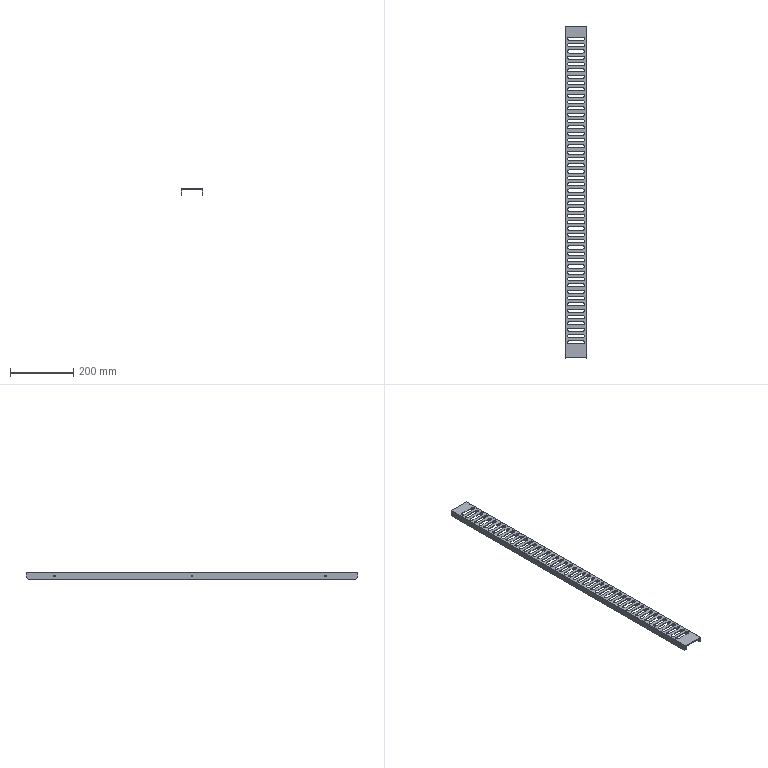Component | SolidWorks | WireDuct2-1 | 1 solid | 271 faces | box 68 x 1050 x 20 mm | volume 168161 mm3 | cylinder 163 | plane 108 | commonest cylinder face diameters 9.991 x147 6 x12 20 x4
build123d program:
from build123d import *

# Parameters (mm, degrees)
BOSS_EXTRUDE1_DEPTH       = 525
BOSS_EXTRUDE1_DEPTH_BACK  = 525
SIZE_MM_DOWEL_PIN_HOLE1_D = 6
FILLET1_R                 = 10
CUT_EXTRUDE1_DEPTH        = 10


with BuildPart() as part:
    # Sketch1 → Boss-Extrude1 (new, two sides: drawn at the far end of the back side and taken through both)
    with BuildSketch(Plane(origin=(0, 0, 0), x_dir=(1, 0, 0), z_dir=(0, 1, 0)).offset(-BOSS_EXTRUDE1_DEPTH_BACK)):
        Polygon((32, 10), (32, -8), (-32, -8), (-32, 10), (-34, 10), (-34, -10), (34, -10), (34, 10), align=None)
    extrude(amount=BOSS_EXTRUDE1_DEPTH + BOSS_EXTRUDE1_DEPTH_BACK)

    # Size mm Dowel Pin Hole1 (through all)
    with Locations(Plane(origin=(34, 0, 0), x_dir=(0, 0, -1), z_dir=(1, 0, 0))):
        with Locations((0, 435.363), (0, 0), (0, -423.324)):
            Hole(SIZE_MM_DOWEL_PIN_HOLE1_D / 2)

    # Fillet1
    fillet1_edges = [part.edges().sort_by_distance(p)[0] for p in [
        (-33, -525, -10),
        (33, 525, -10),
        (-33, 525, -10),
        (33, -525, -10),
    ]]
    fillet(fillet1_edges, radius=FILLET1_R)

    # Sketch5 → Cut-Extrude1 (cut)
    with BuildSketch(Plane.XY.offset(10)):
        with BuildLine():
            Line((-21.471, 489.584), (21.471, 489.584))
            ThreePointArc((21.471, 489.584), (26.467, 484.588), (21.471, 479.593))
            Line((21.471, 479.593), (-21.471, 479.593))
            ThreePointArc((-21.471, 479.593), (-26.467, 484.588), (-21.471, 489.584))
        make_face()
        with BuildLine():
            Line((-21.471, 469.584), (21.471, 469.584))
            ThreePointArc((21.471, 469.584), (26.467, 464.588), (21.471, 459.593))
            Line((21.471, 459.593), (-21.471, 459.593))
            ThreePointArc((-21.471, 459.593), (-26.467, 464.588), (-21.471, 469.584))
        make_face()
        with BuildLine():
            Line((-21.471, 449.584), (21.471, 449.584))
            ThreePointArc((21.471, 449.584), (26.467, 444.588), (21.471, 439.593))
            Line((21.471, 439.593), (-21.471, 439.593))
            ThreePointArc((-21.471, 439.593), (-26.467, 444.588), (-21.471, 449.584))
        make_face()
        with BuildLine():
            Line((-21.471, 429.584), (21.471, 429.584))
            ThreePointArc((21.471, 429.584), (26.467, 424.588), (21.471, 419.593))
            Line((21.471, 419.593), (-21.471, 419.593))
            ThreePointArc((-21.471, 419.593), (-26.467, 424.588), (-21.471, 429.584))
        make_face()
        with BuildLine():
            Line((-21.471, 409.584), (21.471, 409.584))
            ThreePointArc((21.471, 409.584), (26.467, 404.588), (21.471, 399.593))
            Line((21.471, 399.593), (-21.471, 399.593))
            ThreePointArc((-21.471, 399.593), (-26.467, 404.588), (-21.471, 409.584))
        make_face()
        with BuildLine():
            Line((-21.471, 389.584), (21.471, 389.584))
            ThreePointArc((21.471, 389.584), (26.467, 384.588), (21.471, 379.593))
            Line((21.471, 379.593), (-21.471, 379.593))
            ThreePointArc((-21.471, 379.593), (-26.467, 384.588), (-21.471, 389.584))
        make_face()
        with BuildLine():
            Line((-21.471, 369.584), (21.471, 369.584))
            ThreePointArc((21.471, 369.584), (26.467, 364.588), (21.471, 359.593))
            Line((21.471, 359.593), (-21.471, 359.593))
            ThreePointArc((-21.471, 359.593), (-26.467, 364.588), (-21.471, 369.584))
        make_face()
        with BuildLine():
            Line((-21.471, 349.584), (21.471, 349.584))
            ThreePointArc((21.471, 349.584), (26.467, 344.588), (21.471, 339.593))
            Line((21.471, 339.593), (-21.471, 339.593))
            ThreePointArc((-21.471, 339.593), (-26.467, 344.588), (-21.471, 349.584))
        make_face()
        with BuildLine():
            Line((-21.471, 329.584), (21.471, 329.584))
            ThreePointArc((21.471, 329.584), (26.467, 324.588), (21.471, 319.593))
            Line((21.471, 319.593), (-21.471, 319.593))
            ThreePointArc((-21.471, 319.593), (-26.467, 324.588), (-21.471, 329.584))
        make_face()
        with BuildLine():
            Line((-21.471, 309.584), (21.471, 309.584))
            ThreePointArc((21.471, 309.584), (26.467, 304.588), (21.471, 299.593))
            Line((21.471, 299.593), (-21.471, 299.593))
            ThreePointArc((-21.471, 299.593), (-26.467, 304.588), (-21.471, 309.584))
        make_face()
        with BuildLine():
            Line((-21.471, 289.584), (21.471, 289.584))
            ThreePointArc((21.471, 289.584), (26.467, 284.588), (21.471, 279.593))
            Line((21.471, 279.593), (-21.471, 279.593))
            ThreePointArc((-21.471, 279.593), (-26.467, 284.588), (-21.471, 289.584))
        make_face()
        with BuildLine():
            Line((-21.471, 269.584), (21.471, 269.584))
            ThreePointArc((21.471, 269.584), (26.467, 264.588), (21.471, 259.593))
            Line((21.471, 259.593), (-21.471, 259.593))
            ThreePointArc((-21.471, 259.593), (-26.467, 264.588), (-21.471, 269.584))
        make_face()
        with BuildLine():
            Line((-21.471, 249.584), (21.471, 249.584))
            ThreePointArc((21.471, 249.584), (26.467, 244.588), (21.471, 239.593))
            Line((21.471, 239.593), (-21.471, 239.593))
            ThreePointArc((-21.471, 239.593), (-26.467, 244.588), (-21.471, 249.584))
        make_face()
        with BuildLine():
            Line((-21.471, 229.584), (21.471, 229.584))
            ThreePointArc((21.471, 229.584), (26.467, 224.588), (21.471, 219.593))
            Line((21.471, 219.593), (-21.471, 219.593))
            ThreePointArc((-21.471, 219.593), (-26.467, 224.588), (-21.471, 229.584))
        make_face()
        with BuildLine():
            Line((-21.471, 209.584), (21.471, 209.584))
            ThreePointArc((21.471, 209.584), (26.467, 204.588), (21.471, 199.593))
            Line((21.471, 199.593), (-21.471, 199.593))
            ThreePointArc((-21.471, 199.593), (-26.467, 204.588), (-21.471, 209.584))
        make_face()
        with BuildLine():
            Line((-21.471, 189.584), (21.471, 189.584))
            ThreePointArc((21.471, 189.584), (26.467, 184.588), (21.471, 179.593))
            Line((21.471, 179.593), (-21.471, 179.593))
            ThreePointArc((-21.471, 179.593), (-26.467, 184.588), (-21.471, 189.584))
        make_face()
        with BuildLine():
            Line((-21.471, 169.584), (21.471, 169.584))
            ThreePointArc((21.471, 169.584), (26.467, 164.588), (21.471, 159.593))
            Line((21.471, 159.593), (-21.471, 159.593))
            ThreePointArc((-21.471, 159.593), (-26.467, 164.588), (-21.471, 169.584))
        make_face()
        with BuildLine():
            Line((-21.471, 149.584), (21.471, 149.584))
            ThreePointArc((21.471, 149.584), (26.467, 144.588), (21.471, 139.593))
            Line((21.471, 139.593), (-21.471, 139.593))
            ThreePointArc((-21.471, 139.593), (-26.467, 144.588), (-21.471, 149.584))
        make_face()
        with BuildLine():
            Line((-21.471, 129.584), (21.471, 129.584))
            ThreePointArc((21.471, 129.584), (26.467, 124.588), (21.471, 119.593))
            Line((21.471, 119.593), (-21.471, 119.593))
            ThreePointArc((-21.471, 119.593), (-26.467, 124.588), (-21.471, 129.584))
        make_face()
        with BuildLine():
            Line((-21.471, 109.584), (21.471, 109.584))
            ThreePointArc((21.471, 109.584), (26.467, 104.588), (21.471, 99.593))
            Line((21.471, 99.593), (-21.471, 99.593))
            ThreePointArc((-21.471, 99.593), (-26.467, 104.588), (-21.471, 109.584))
        make_face()
        with BuildLine():
            Line((-21.471, 89.584), (21.471, 89.584))
            ThreePointArc((21.471, 89.584), (26.467, 84.588), (21.471, 79.593))
            Line((21.471, 79.593), (-21.471, 79.593))
            ThreePointArc((-21.471, 79.593), (-26.467, 84.588), (-21.471, 89.584))
        make_face()
        with BuildLine():
            Line((-21.471, 69.584), (21.471, 69.584))
            ThreePointArc((21.471, 69.584), (26.467, 64.588), (21.471, 59.593))
            Line((21.471, 59.593), (-21.471, 59.593))
            ThreePointArc((-21.471, 59.593), (-26.467, 64.588), (-21.471, 69.584))
        make_face()
        with BuildLine():
            Line((-21.471, 49.584), (21.471, 49.584))
            ThreePointArc((21.471, 49.584), (26.467, 44.588), (21.471, 39.593))
            Line((21.471, 39.593), (-21.471, 39.593))
            ThreePointArc((-21.471, 39.593), (-26.467, 44.588), (-21.471, 49.584))
        make_face()
        with BuildLine():
            Line((-21.471, 29.584), (21.471, 29.584))
            ThreePointArc((21.471, 29.584), (26.467, 24.588), (21.471, 19.593))
            Line((21.471, 19.593), (-21.471, 19.593))
            ThreePointArc((-21.471, 19.593), (-26.467, 24.588), (-21.471, 29.584))
        make_face()
        with BuildLine():
            Line((-21.471, 9.584), (21.471, 9.584))
            ThreePointArc((21.471, 9.584), (26.467, 4.588), (21.471, -0.4072))
            Line((21.471, -0.4072), (-21.471, -0.4072))
            ThreePointArc((-21.471, -0.4072), (-26.467, 4.588), (-21.471, 9.584))
        make_face()
        with BuildLine():
            Line((-21.471, -10.416), (21.471, -10.416))
            ThreePointArc((21.471, -10.416), (26.467, -15.412), (21.471, -20.407))
            Line((21.471, -20.407), (-21.471, -20.407))
            ThreePointArc((-21.471, -20.407), (-26.467, -15.412), (-21.471, -10.416))
        make_face()
        with BuildLine():
            Line((-21.471, -30.416), (21.471, -30.416))
            ThreePointArc((21.471, -30.416), (26.467, -35.412), (21.471, -40.407))
            Line((21.471, -40.407), (-21.471, -40.407))
            ThreePointArc((-21.471, -40.407), (-26.467, -35.412), (-21.471, -30.416))
        make_face()
        with BuildLine():
            Line((-21.471, -50.416), (21.471, -50.416))
            ThreePointArc((21.471, -50.416), (26.467, -55.412), (21.471, -60.407))
            Line((21.471, -60.407), (-21.471, -60.407))
            ThreePointArc((-21.471, -60.407), (-26.467, -55.412), (-21.471, -50.416))
        make_face()
        with BuildLine():
            Line((-21.471, -70.416), (21.471, -70.416))
            ThreePointArc((21.471, -70.416), (26.467, -75.412), (21.471, -80.407))
            Line((21.471, -80.407), (-21.471, -80.407))
            ThreePointArc((-21.471, -80.407), (-26.467, -75.412), (-21.471, -70.416))
        make_face()
        with BuildLine():
            Line((-21.471, -90.416), (21.471, -90.416))
            ThreePointArc((21.471, -90.416), (26.467, -95.412), (21.471, -100.407))
            Line((21.471, -100.407), (-21.471, -100.407))
            ThreePointArc((-21.471, -100.407), (-26.467, -95.412), (-21.471, -90.416))
        make_face()
        with BuildLine():
            Line((-21.471, -110.416), (21.471, -110.416))
            ThreePointArc((21.471, -110.416), (26.467, -115.412), (21.471, -120.407))
            Line((21.471, -120.407), (-21.471, -120.407))
            ThreePointArc((-21.471, -120.407), (-26.467, -115.412), (-21.471, -110.416))
        make_face()
        with BuildLine():
            Line((-21.471, -130.416), (21.471, -130.416))
            ThreePointArc((21.471, -130.416), (26.467, -135.412), (21.471, -140.407))
            Line((21.471, -140.407), (-21.471, -140.407))
            ThreePointArc((-21.471, -140.407), (-26.467, -135.412), (-21.471, -130.416))
        make_face()
        with BuildLine():
            Line((-21.471, -150.416), (21.471, -150.416))
            ThreePointArc((21.471, -150.416), (26.467, -155.412), (21.471, -160.407))
            Line((21.471, -160.407), (-21.471, -160.407))
            ThreePointArc((-21.471, -160.407), (-26.467, -155.412), (-21.471, -150.416))
        make_face()
        with BuildLine():
            Line((-21.471, -170.416), (21.471, -170.416))
            ThreePointArc((21.471, -170.416), (26.467, -175.412), (21.471, -180.407))
            Line((21.471, -180.407), (-21.471, -180.407))
            ThreePointArc((-21.471, -180.407), (-26.467, -175.412), (-21.471, -170.416))
        make_face()
        with BuildLine():
            Line((-21.471, -190.416), (21.471, -190.416))
            ThreePointArc((21.471, -190.416), (26.467, -195.412), (21.471, -200.407))
            Line((21.471, -200.407), (-21.471, -200.407))
            ThreePointArc((-21.471, -200.407), (-26.467, -195.412), (-21.471, -190.416))
        make_face()
        with BuildLine():
            Line((-21.471, -210.416), (21.471, -210.416))
            ThreePointArc((21.471, -210.416), (26.467, -215.412), (21.471, -220.407))
            Line((21.471, -220.407), (-21.471, -220.407))
            ThreePointArc((-21.471, -220.407), (-26.467, -215.412), (-21.471, -210.416))
        make_face()
        with BuildLine():
            Line((-21.471, -230.416), (21.471, -230.416))
            ThreePointArc((21.471, -230.416), (26.467, -235.412), (21.471, -240.407))
            Line((21.471, -240.407), (-21.471, -240.407))
            ThreePointArc((-21.471, -240.407), (-26.467, -235.412), (-21.471, -230.416))
        make_face()
        with BuildLine():
            Line((-21.471, -250.416), (21.471, -250.416))
            ThreePointArc((21.471, -250.416), (26.467, -255.412), (21.471, -260.407))
            Line((21.471, -260.407), (-21.471, -260.407))
            ThreePointArc((-21.471, -260.407), (-26.467, -255.412), (-21.471, -250.416))
        make_face()
        with BuildLine():
            Line((-21.471, -270.416), (21.471, -270.416))
            ThreePointArc((21.471, -270.416), (26.467, -275.412), (21.471, -280.407))
            Line((21.471, -280.407), (-21.471, -280.407))
            ThreePointArc((-21.471, -280.407), (-26.467, -275.412), (-21.471, -270.416))
        make_face()
        with BuildLine():
            Line((-21.471, -290.416), (21.471, -290.416))
            ThreePointArc((21.471, -290.416), (26.467, -295.412), (21.471, -300.407))
            Line((21.471, -300.407), (-21.471, -300.407))
            ThreePointArc((-21.471, -300.407), (-26.467, -295.412), (-21.471, -290.416))
        make_face()
        with BuildLine():
            Line((-21.471, -310.416), (21.471, -310.416))
            ThreePointArc((21.471, -310.416), (26.467, -315.412), (21.471, -320.407))
            Line((21.471, -320.407), (-21.471, -320.407))
            ThreePointArc((-21.471, -320.407), (-26.467, -315.412), (-21.471, -310.416))
        make_face()
        with BuildLine():
            Line((-21.471, -330.416), (21.471, -330.416))
            ThreePointArc((21.471, -330.416), (26.467, -335.412), (21.471, -340.407))
            Line((21.471, -340.407), (-21.471, -340.407))
            ThreePointArc((-21.471, -340.407), (-26.467, -335.412), (-21.471, -330.416))
        make_face()
        with BuildLine():
            Line((-21.471, -350.416), (21.471, -350.416))
            ThreePointArc((21.471, -350.416), (26.467, -355.412), (21.471, -360.407))
            Line((21.471, -360.407), (-21.471, -360.407))
            ThreePointArc((-21.471, -360.407), (-26.467, -355.412), (-21.471, -350.416))
        make_face()
        with BuildLine():
            Line((-21.471, -370.416), (21.471, -370.416))
            ThreePointArc((21.471, -370.416), (26.467, -375.412), (21.471, -380.407))
            Line((21.471, -380.407), (-21.471, -380.407))
            ThreePointArc((-21.471, -380.407), (-26.467, -375.412), (-21.471, -370.416))
        make_face()
        with BuildLine():
            Line((-21.471, -390.416), (21.471, -390.416))
            ThreePointArc((21.471, -390.416), (26.467, -395.412), (21.471, -400.407))
            Line((21.471, -400.407), (-21.471, -400.407))
            ThreePointArc((-21.471, -400.407), (-26.467, -395.412), (-21.471, -390.416))
        make_face()
        with BuildLine():
            Line((-21.471, -410.416), (21.471, -410.416))
            ThreePointArc((21.471, -410.416), (26.467, -415.412), (21.471, -420.407))
            Line((21.471, -420.407), (-21.471, -420.407))
            ThreePointArc((-21.471, -420.407), (-26.467, -415.412), (-21.471, -410.416))
        make_face()
        with BuildLine():
            Line((-21.471, -430.416), (21.471, -430.416))
            ThreePointArc((21.471, -430.416), (26.467, -435.412), (21.471, -440.407))
            Line((21.471, -440.407), (-21.471, -440.407))
            ThreePointArc((-21.471, -440.407), (-26.467, -435.412), (-21.471, -430.416))
        make_face()
        with BuildLine():
            Line((-21.471, -450.416), (21.471, -450.416))
            ThreePointArc((21.471, -450.416), (26.467, -455.412), (21.471, -460.407))
            Line((21.471, -460.407), (-21.471, -460.407))
            ThreePointArc((-21.471, -460.407), (-26.467, -455.412), (-21.471, -450.416))
        make_face()
        with BuildLine():
            Line((-21.471, -470.416), (21.471, -470.416))
            ThreePointArc((21.471, -470.416), (26.467, -475.412), (21.471, -480.407))
            Line((21.471, -480.407), (-21.471, -480.407))
            ThreePointArc((-21.471, -480.407), (-26.467, -475.412), (-21.471, -470.416))
        make_face()
    extrude(amount=-CUT_EXTRUDE1_DEPTH, mode=Mode.SUBTRACT)


solid = part.part

# Placed as in the assembly
solid = solid.moved(Location((613, 1495, -2111), (0, 0, 0)))